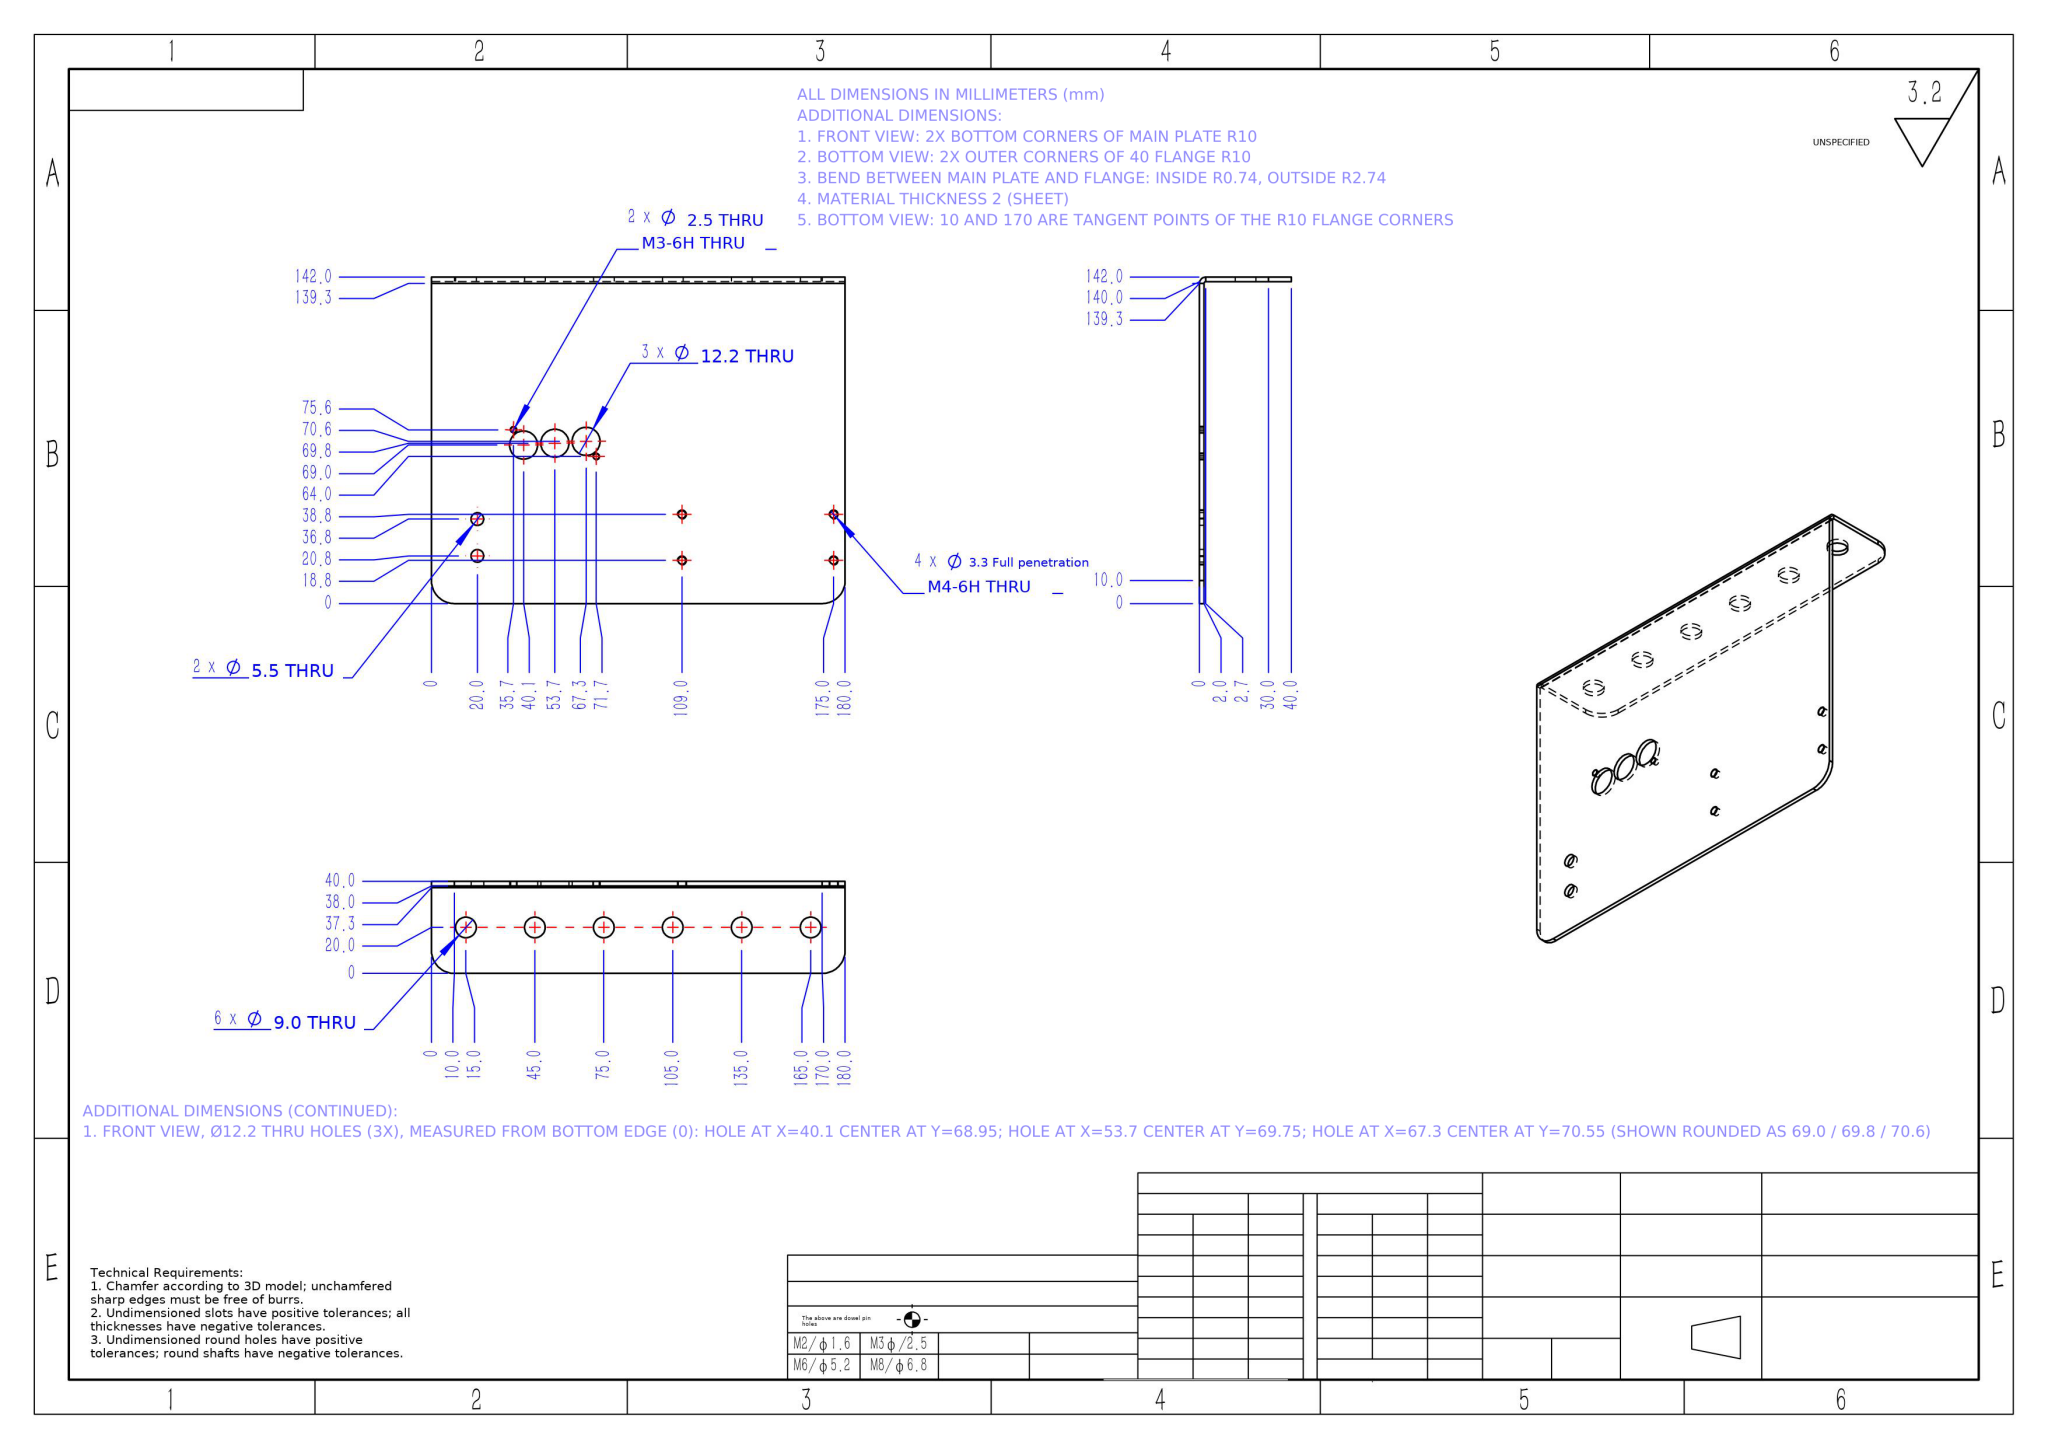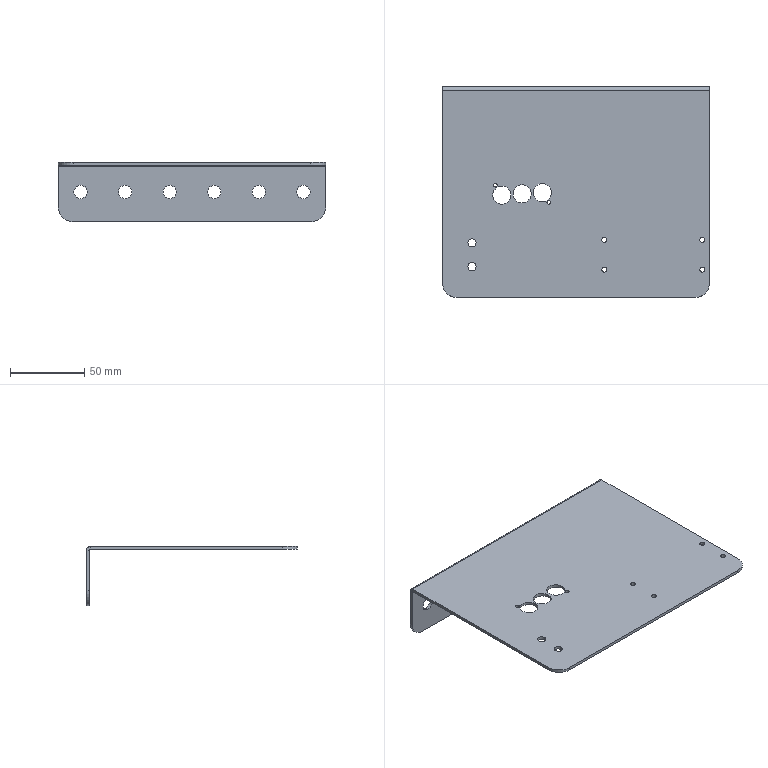Part | NX | mm | 1 solid | 52 faces | box 180 x 142 x 40 mm | volume 62712 mm3 | cylinder 40 | plane 12 | commonest cylinder face diameters 9 x12 3.3 x8 12.2 x6 2.5 x4 5.5 x4 20 x4 5.473 x1 1.473 x1